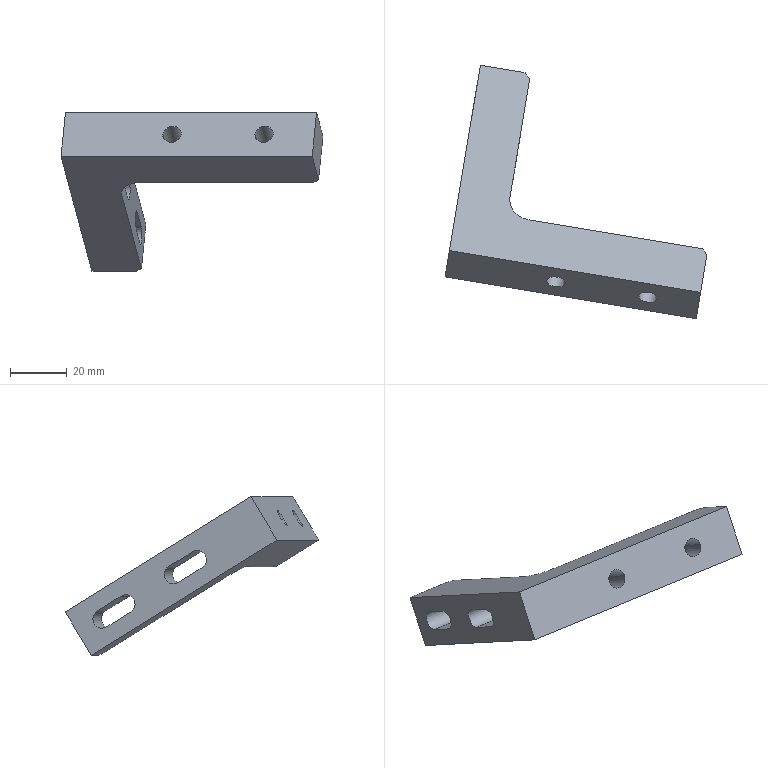Component | SolidWorks | 14AC-24-1-008-1 | 1 solid | 31 faces | box 92.56 x 89.67 x 56.08 mm | volume 43107 mm3 | plane 16 | cylinder 14 | spline 1 | commonest cylinder face diameters 6.6 x8 11 x4 16 x2
STEP:
#1=COLOUR_RGB('',0.7922,0.8196,0.9333);
#2=FILL_AREA_STYLE_COLOUR('',#1);
#3=FILL_AREA_STYLE('',(#2));
#4=SURFACE_STYLE_FILL_AREA(#3);
#5=SURFACE_SIDE_STYLE('',(#4));
#6=SURFACE_STYLE_USAGE(.BOTH.,#5);
#7=PRESENTATION_STYLE_ASSIGNMENT((#6));
#8=CARTESIAN_POINT('',(19.576,-9.025,-4.805));
#9=VERTEX_POINT('',#8);
#10=CARTESIAN_POINT('',(19.149,-8.954,-4.805));
#11=VERTEX_POINT('',#10);
#12=CARTESIAN_POINT('',(19.362,-8.99,-4.805));
#13=DIRECTION('',(0.1401,0.8413,-0.5222));
#14=DIRECTION('',(-0.9864,0.1642,0.));
#15=AXIS2_PLACEMENT_3D('',#12,#13,#14);
#16=CIRCLE('',#15,0.2165);
#17=EDGE_CURVE('',#9,#11,#16,.T.);
#18=ORIENTED_EDGE('',*,*,#17,.F.);
#19=CARTESIAN_POINT('',(19.613,-8.8,-4.944));
#20=VERTEX_POINT('',#19);
#21=CARTESIAN_POINT('',(19.613,-8.8,-4.944));
#22=DIRECTION('',(0.1401,0.8413,-0.5222));
#23=VECTOR('',#22,39.37);
#24=LINE('',#21,#23);
#25=EDGE_CURVE('',#9,#20,#24,.T.);
#26=ORIENTED_EDGE('',*,*,#25,.T.);
#27=CARTESIAN_POINT('',(19.186,-8.729,-4.944));
#28=VERTEX_POINT('',#27);
#29=CARTESIAN_POINT('',(19.4,-8.765,-4.944));
#30=DIRECTION('',(0.1401,0.8413,-0.5222));
#31=DIRECTION('',(-0.9864,0.1642,0.));
#32=AXIS2_PLACEMENT_3D('',#29,#30,#31);
#33=CIRCLE('',#32,0.2165);
#34=EDGE_CURVE('',#20,#28,#33,.T.);
#35=ORIENTED_EDGE('',*,*,#34,.T.);
#36=CARTESIAN_POINT('',(19.186,-8.729,-4.944));
#37=DIRECTION('',(0.1401,0.8413,-0.5222));
#38=VECTOR('',#37,39.37);
#39=LINE('',#36,#38);
#40=EDGE_CURVE('',#11,#28,#39,.T.);
#41=ORIENTED_EDGE('',*,*,#40,.F.);
#42=EDGE_LOOP('',(#18,#26,#35,#41));
#43=FACE_OUTER_BOUND('',#42,.T.);
#44=CARTESIAN_POINT('',(19.4,-8.765,-4.944));
#45=DIRECTION('',(0.1401,0.8413,-0.5222));
#46=DIRECTION('',(-0.9864,0.1642,0.));
#47=AXIS2_PLACEMENT_3D('',#44,#45,#46);
#48=CYLINDRICAL_SURFACE('',#47,0.2165);
#49=ADVANCED_FACE('',(#43),#48,.F.);
#50=CARTESIAN_POINT('',(19.429,-9.382,-4.574));
#51=VERTEX_POINT('',#50);
#52=CARTESIAN_POINT('',(19.172,-9.34,-4.574));
#53=VERTEX_POINT('',#52);
#54=CARTESIAN_POINT('',(19.301,-9.361,-4.574));
#55=DIRECTION('',(0.1401,0.8413,-0.5222));
#56=DIRECTION('',(-0.9864,0.1642,0.));
#57=AXIS2_PLACEMENT_3D('',#54,#55,#56);
#58=CIRCLE('',#57,0.1299);
#59=EDGE_CURVE('',#51,#53,#58,.T.);
#60=ORIENTED_EDGE('',*,*,#59,.F.);
#61=CARTESIAN_POINT('',(19.49,-9.011,-4.805));
#62=VERTEX_POINT('',#61);
#63=CARTESIAN_POINT('',(19.528,-8.786,-4.944));
#64=DIRECTION('',(0.1401,0.8413,-0.5222));
#65=VECTOR('',#64,39.37);
#66=LINE('',#63,#65);
#67=EDGE_CURVE('',#51,#62,#66,.T.);
#68=ORIENTED_EDGE('',*,*,#67,.T.);
#69=CARTESIAN_POINT('',(19.234,-8.969,-4.805));
#70=VERTEX_POINT('',#69);
#71=CARTESIAN_POINT('',(19.362,-8.99,-4.805));
#72=DIRECTION('',(0.1401,0.8413,-0.5222));
#73=DIRECTION('',(-0.9864,0.1642,0.));
#74=AXIS2_PLACEMENT_3D('',#71,#72,#73);
#75=CIRCLE('',#74,0.1299);
#76=EDGE_CURVE('',#62,#70,#75,.T.);
#77=ORIENTED_EDGE('',*,*,#76,.T.);
#78=CARTESIAN_POINT('',(19.272,-8.743,-4.944));
#79=DIRECTION('',(0.1401,0.8413,-0.5222));
#80=VECTOR('',#79,39.37);
#81=LINE('',#78,#80);
#82=EDGE_CURVE('',#53,#70,#81,.T.);
#83=ORIENTED_EDGE('',*,*,#82,.F.);
#84=EDGE_LOOP('',(#60,#68,#77,#83));
#85=FACE_OUTER_BOUND('',#84,.T.);
#86=CARTESIAN_POINT('',(19.4,-8.765,-4.944));
#87=DIRECTION('',(0.1401,0.8413,-0.5222));
#88=DIRECTION('',(-0.9864,0.1642,0.));
#89=AXIS2_PLACEMENT_3D('',#86,#87,#88);
#90=CYLINDRICAL_SURFACE('',#89,0.1299);
#91=ADVANCED_FACE('',(#85),#90,.F.);
#92=CARTESIAN_POINT('',(18.294,-8.812,-4.805));
#93=VERTEX_POINT('',#92);
#94=CARTESIAN_POINT('',(17.867,-8.741,-4.805));
#95=VERTEX_POINT('',#94);
#96=CARTESIAN_POINT('',(18.081,-8.776,-4.805));
#97=DIRECTION('',(0.1401,0.8413,-0.5222));
#98=DIRECTION('',(-0.9864,0.1642,0.));
#99=AXIS2_PLACEMENT_3D('',#96,#97,#98);
#100=CIRCLE('',#99,0.2165);
#101=EDGE_CURVE('',#93,#95,#100,.T.);
#102=ORIENTED_EDGE('',*,*,#101,.F.);
#103=CARTESIAN_POINT('',(18.332,-8.587,-4.944));
#104=VERTEX_POINT('',#103);
#105=CARTESIAN_POINT('',(18.332,-8.587,-4.944));
#106=DIRECTION('',(0.1401,0.8413,-0.5222));
#107=VECTOR('',#106,39.37);
#108=LINE('',#105,#107);
#109=EDGE_CURVE('',#93,#104,#108,.T.);
#110=ORIENTED_EDGE('',*,*,#109,.T.);
#111=CARTESIAN_POINT('',(17.905,-8.516,-4.944));
#112=VERTEX_POINT('',#111);
#113=CARTESIAN_POINT('',(18.118,-8.551,-4.944));
#114=DIRECTION('',(0.1401,0.8413,-0.5222));
#115=DIRECTION('',(-0.9864,0.1642,0.));
#116=AXIS2_PLACEMENT_3D('',#113,#114,#115);
#117=CIRCLE('',#116,0.2165);
#118=EDGE_CURVE('',#104,#112,#117,.T.);
#119=ORIENTED_EDGE('',*,*,#118,.T.);
#120=CARTESIAN_POINT('',(17.905,-8.516,-4.944));
#121=DIRECTION('',(0.1401,0.8413,-0.5222));
#122=VECTOR('',#121,39.37);
#123=LINE('',#120,#122);
#124=EDGE_CURVE('',#95,#112,#123,.T.);
#125=ORIENTED_EDGE('',*,*,#124,.F.);
#126=EDGE_LOOP('',(#102,#110,#119,#125));
#127=FACE_OUTER_BOUND('',#126,.T.);
#128=CARTESIAN_POINT('',(18.118,-8.551,-4.944));
#129=DIRECTION('',(0.1401,0.8413,-0.5222));
#130=DIRECTION('',(-0.9864,0.1642,0.));
#131=AXIS2_PLACEMENT_3D('',#128,#129,#130);
#132=CYLINDRICAL_SURFACE('',#131,0.2165);
#133=ADVANCED_FACE('',(#127),#132,.F.);
#134=CARTESIAN_POINT('',(18.147,-9.169,-4.574));
#135=VERTEX_POINT('',#134);
#136=CARTESIAN_POINT('',(17.891,-9.126,-4.574));
#137=VERTEX_POINT('',#136);
#138=CARTESIAN_POINT('',(18.019,-9.147,-4.574));
#139=DIRECTION('',(0.1401,0.8413,-0.5222));
#140=DIRECTION('',(-0.9864,0.1642,0.));
#141=AXIS2_PLACEMENT_3D('',#138,#139,#140);
#142=CIRCLE('',#141,0.1299);
#143=EDGE_CURVE('',#135,#137,#142,.T.);
#144=ORIENTED_EDGE('',*,*,#143,.F.);
#145=CARTESIAN_POINT('',(18.209,-8.798,-4.805));
#146=VERTEX_POINT('',#145);
#147=CARTESIAN_POINT('',(18.246,-8.573,-4.944));
#148=DIRECTION('',(0.1401,0.8413,-0.5222));
#149=VECTOR('',#148,39.37);
#150=LINE('',#147,#149);
#151=EDGE_CURVE('',#135,#146,#150,.T.);
#152=ORIENTED_EDGE('',*,*,#151,.T.);
#153=CARTESIAN_POINT('',(17.953,-8.755,-4.805));
#154=VERTEX_POINT('',#153);
#155=CARTESIAN_POINT('',(18.081,-8.776,-4.805));
#156=DIRECTION('',(0.1401,0.8413,-0.5222));
#157=DIRECTION('',(-0.9864,0.1642,0.));
#158=AXIS2_PLACEMENT_3D('',#155,#156,#157);
#159=CIRCLE('',#158,0.1299);
#160=EDGE_CURVE('',#146,#154,#159,.T.);
#161=ORIENTED_EDGE('',*,*,#160,.T.);
#162=CARTESIAN_POINT('',(17.99,-8.53,-4.944));
#163=DIRECTION('',(0.1401,0.8413,-0.5222));
#164=VECTOR('',#163,39.37);
#165=LINE('',#162,#164);
#166=EDGE_CURVE('',#137,#154,#165,.T.);
#167=ORIENTED_EDGE('',*,*,#166,.F.);
#168=EDGE_LOOP('',(#144,#152,#161,#167));
#169=FACE_OUTER_BOUND('',#168,.T.);
#170=CARTESIAN_POINT('',(18.118,-8.551,-4.944));
#171=DIRECTION('',(0.1401,0.8413,-0.5222));
#172=DIRECTION('',(-0.9864,0.1642,0.));
#173=AXIS2_PLACEMENT_3D('',#170,#171,#172);
#174=CYLINDRICAL_SURFACE('',#173,0.1299);
#175=ADVANCED_FACE('',(#169),#174,.F.);
#176=CARTESIAN_POINT('',(17.526,-6.598,-6.48));
#177=VERTEX_POINT('',#176);
#178=CARTESIAN_POINT('',(16.904,-6.494,-6.48));
#179=VERTEX_POINT('',#178);
#180=CARTESIAN_POINT('',(20.399,-7.076,-6.48));
#181=DIRECTION('',(-0.9864,0.1642,-0.));
#182=VECTOR('',#181,39.37);
#183=LINE('',#180,#182);
#184=EDGE_CURVE('',#177,#179,#183,.T.);
#185=ORIENTED_EDGE('',*,*,#184,.F.);
#186=CARTESIAN_POINT('',(17.592,-6.677,-6.439));
#187=VERTEX_POINT('',#186);
#188=CARTESIAN_POINT('',(17.526,-6.598,-6.48));
#189=DIRECTION('',(0.5985,-0.711,0.3692));
#190=VECTOR('',#189,39.37);
#191=LINE('',#188,#190);
#192=EDGE_CURVE('',#177,#187,#191,.T.);
#193=ORIENTED_EDGE('',*,*,#192,.T.);
#194=CARTESIAN_POINT('',(17.316,-8.333,-5.411));
#195=VERTEX_POINT('',#194);
#196=CARTESIAN_POINT('',(17.603,-6.611,-6.48));
#197=DIRECTION('',(0.1401,0.8413,-0.5222));
#198=VECTOR('',#197,39.37);
#199=LINE('',#196,#198);
#200=EDGE_CURVE('',#195,#187,#199,.T.);
#201=ORIENTED_EDGE('',*,*,#200,.F.);
#202=CARTESIAN_POINT('',(17.583,-8.65,-5.247));
#203=VERTEX_POINT('',#202);
#204=CARTESIAN_POINT('',(17.627,-8.385,-5.411));
#205=DIRECTION('',(0.08576,0.5151,0.8529));
#206=DIRECTION('',(-0.9864,0.1642,0.));
#207=AXIS2_PLACEMENT_3D('',#204,#205,#206);
#208=CIRCLE('',#207,0.315);
#209=EDGE_CURVE('',#195,#203,#208,.T.);
#210=ORIENTED_EDGE('',*,*,#209,.T.);
#211=CARTESIAN_POINT('',(19.991,-9.051,-5.247));
#212=VERTEX_POINT('',#211);
#213=CARTESIAN_POINT('',(20.068,-9.064,-5.247));
#214=DIRECTION('',(-0.9864,0.1642,-0.));
#215=VECTOR('',#214,39.37);
#216=LINE('',#213,#215);
#217=EDGE_CURVE('',#212,#203,#216,.T.);
#218=ORIENTED_EDGE('',*,*,#217,.F.);
#219=CARTESIAN_POINT('',(20.057,-9.13,-5.205));
#220=VERTEX_POINT('',#219);
#221=CARTESIAN_POINT('',(19.991,-9.051,-5.247));
#222=DIRECTION('',(0.5985,-0.711,0.3692));
#223=VECTOR('',#222,39.37);
#224=LINE('',#221,#223);
#225=EDGE_CURVE('',#212,#220,#224,.T.);
#226=ORIENTED_EDGE('',*,*,#225,.T.);
#227=CARTESIAN_POINT('',(19.969,-9.66,-4.877));
#228=VERTEX_POINT('',#227);
#229=CARTESIAN_POINT('',(20.399,-7.076,-6.48));
#230=DIRECTION('',(0.1401,0.8413,-0.5222));
#231=VECTOR('',#230,39.37);
#232=LINE('',#229,#231);
#233=EDGE_CURVE('',#228,#220,#232,.T.);
#234=ORIENTED_EDGE('',*,*,#233,.F.);
#235=CARTESIAN_POINT('',(16.474,-9.078,-4.877));
#236=VERTEX_POINT('',#235);
#237=CARTESIAN_POINT('',(19.969,-9.66,-4.877));
#238=DIRECTION('',(-0.9864,0.1642,-0.));
#239=VECTOR('',#238,39.37);
#240=LINE('',#237,#239);
#241=EDGE_CURVE('',#228,#236,#240,.T.);
#242=ORIENTED_EDGE('',*,*,#241,.T.);
#243=CARTESIAN_POINT('',(16.904,-6.494,-6.48));
#244=DIRECTION('',(0.1401,0.8413,-0.5222));
#245=VECTOR('',#244,39.37);
#246=LINE('',#243,#245);
#247=EDGE_CURVE('',#236,#179,#246,.T.);
#248=ORIENTED_EDGE('',*,*,#247,.T.);
#249=EDGE_LOOP('',(#185,#193,#201,#210,#218,#226,#234,#242,#248));
#250=FACE_OUTER_BOUND('',#249,.T.);
#251=CARTESIAN_POINT('',(20.399,-7.076,-6.48));
#252=DIRECTION('',(0.08576,0.5151,0.8529));
#253=DIRECTION('',(-0.9864,0.1642,-0.));
#254=AXIS2_PLACEMENT_3D('',#251,#252,#253);
#255=PLANE('',#254);
#256=ADVANCED_FACE('',(#250),#255,.F.);
#257=CARTESIAN_POINT('',(17.586,-6.233,-5.876));
#258=VERTEX_POINT('',#257);
#259=CARTESIAN_POINT('',(16.965,-6.129,-5.876));
#260=VERTEX_POINT('',#259);
#261=CARTESIAN_POINT('',(20.46,-6.711,-5.876));
#262=DIRECTION('',(-0.9864,0.1642,-0.));
#263=VECTOR('',#262,39.37);
#264=LINE('',#261,#263);
#265=EDGE_CURVE('',#258,#260,#264,.T.);
#266=ORIENTED_EDGE('',*,*,#265,.F.);
#267=CARTESIAN_POINT('',(17.526,-6.598,-6.48));
#268=DIRECTION('',(-0.08576,-0.5151,-0.8529));
#269=VECTOR('',#268,39.37);
#270=LINE('',#267,#269);
#271=EDGE_CURVE('',#258,#177,#270,.T.);
#272=ORIENTED_EDGE('',*,*,#271,.T.);
#273=ORIENTED_EDGE('',*,*,#184,.T.);
#274=CARTESIAN_POINT('',(16.904,-6.494,-6.48));
#275=DIRECTION('',(0.08576,0.5151,0.8529));
#276=VECTOR('',#275,39.37);
#277=LINE('',#274,#276);
#278=EDGE_CURVE('',#179,#260,#277,.T.);
#279=ORIENTED_EDGE('',*,*,#278,.T.);
#280=EDGE_LOOP('',(#266,#272,#273,#279));
#281=FACE_OUTER_BOUND('',#280,.T.);
#282=CARTESIAN_POINT('',(20.399,-7.076,-6.48));
#283=DIRECTION('',(-0.1401,-0.8413,0.5222));
#284=DIRECTION('',(0.9864,-0.1642,0.));
#285=AXIS2_PLACEMENT_3D('',#282,#283,#284);
#286=PLANE('',#285);
#287=ADVANCED_FACE('',(#281),#286,.F.);
#288=CARTESIAN_POINT('',(17.377,-7.968,-4.807));
#289=VERTEX_POINT('',#288);
#290=CARTESIAN_POINT('',(17.653,-6.312,-5.835));
#291=VERTEX_POINT('',#290);
#292=CARTESIAN_POINT('',(17.664,-6.246,-5.876));
#293=DIRECTION('',(0.1401,0.8413,-0.5222));
#294=VECTOR('',#293,39.37);
#295=LINE('',#292,#294);
#296=EDGE_CURVE('',#289,#291,#295,.T.);
#297=ORIENTED_EDGE('',*,*,#296,.T.);
#298=CARTESIAN_POINT('',(17.586,-6.233,-5.876));
#299=DIRECTION('',(-0.5985,0.711,-0.3692));
#300=VECTOR('',#299,39.37);
#301=LINE('',#298,#300);
#302=EDGE_CURVE('',#291,#258,#301,.T.);
#303=ORIENTED_EDGE('',*,*,#302,.T.);
#304=ORIENTED_EDGE('',*,*,#265,.T.);
#305=CARTESIAN_POINT('',(16.535,-8.713,-4.272));
#306=VERTEX_POINT('',#305);
#307=CARTESIAN_POINT('',(16.965,-6.129,-5.876));
#308=DIRECTION('',(-0.1401,-0.8413,0.5222));
#309=VECTOR('',#308,39.37);
#310=LINE('',#307,#309);
#311=EDGE_CURVE('',#260,#306,#310,.T.);
#312=ORIENTED_EDGE('',*,*,#311,.T.);
#313=CARTESIAN_POINT('',(20.03,-9.295,-4.272));
#314=VERTEX_POINT('',#313);
#315=CARTESIAN_POINT('',(20.03,-9.295,-4.272));
#316=DIRECTION('',(-0.9864,0.1642,-0.));
#317=VECTOR('',#316,39.37);
#318=LINE('',#315,#317);
#319=EDGE_CURVE('',#314,#306,#318,.T.);
#320=ORIENTED_EDGE('',*,*,#319,.F.);
#321=CARTESIAN_POINT('',(20.118,-8.765,-4.601));
#322=VERTEX_POINT('',#321);
#323=CARTESIAN_POINT('',(20.46,-6.711,-5.876));
#324=DIRECTION('',(-0.1401,-0.8413,0.5222));
#325=VECTOR('',#324,39.37);
#326=LINE('',#323,#325);
#327=EDGE_CURVE('',#322,#314,#326,.T.);
#328=ORIENTED_EDGE('',*,*,#327,.F.);
#329=CARTESIAN_POINT('',(20.052,-8.686,-4.642));
#330=VERTEX_POINT('',#329);
#331=CARTESIAN_POINT('',(20.052,-8.686,-4.642));
#332=DIRECTION('',(-0.5985,0.711,-0.3692));
#333=VECTOR('',#332,39.37);
#334=LINE('',#331,#333);
#335=EDGE_CURVE('',#322,#330,#334,.T.);
#336=ORIENTED_EDGE('',*,*,#335,.T.);
#337=CARTESIAN_POINT('',(17.644,-8.285,-4.642));
#338=VERTEX_POINT('',#337);
#339=CARTESIAN_POINT('',(20.129,-8.699,-4.642));
#340=DIRECTION('',(-0.9864,0.1642,-0.));
#341=VECTOR('',#340,39.37);
#342=LINE('',#339,#341);
#343=EDGE_CURVE('',#330,#338,#342,.T.);
#344=ORIENTED_EDGE('',*,*,#343,.T.);
#345=CARTESIAN_POINT('',(17.688,-8.02,-4.807));
#346=DIRECTION('',(-0.08576,-0.5151,-0.8529));
#347=DIRECTION('',(0.9864,-0.1642,0.));
#348=AXIS2_PLACEMENT_3D('',#345,#346,#347);
#349=CIRCLE('',#348,0.315);
#350=EDGE_CURVE('',#338,#289,#349,.T.);
#351=ORIENTED_EDGE('',*,*,#350,.T.);
#352=EDGE_LOOP('',(#297,#303,#304,#312,#320,#328,#336,#344,#351));
#353=FACE_OUTER_BOUND('',#352,.T.);
#354=CARTESIAN_POINT('',(20.46,-6.711,-5.876));
#355=DIRECTION('',(-0.08576,-0.5151,-0.8529));
#356=DIRECTION('',(0.9864,-0.1642,0.));
#357=AXIS2_PLACEMENT_3D('',#354,#355,#356);
#358=PLANE('',#357);
#359=ADVANCED_FACE('',(#353),#358,.F.);
#360=CARTESIAN_POINT('',(19.301,-9.361,-4.574));
#361=DIRECTION('',(0.1401,0.8413,-0.5222));
#362=DIRECTION('',(-0.9864,0.1642,0.));
#363=AXIS2_PLACEMENT_3D('',#360,#361,#362);
#364=CIRCLE('',#363,0.1299);
#365=EDGE_CURVE('',#53,#51,#364,.T.);
#366=ORIENTED_EDGE('',*,*,#365,.T.);
#367=ORIENTED_EDGE('',*,*,#59,.T.);
#368=EDGE_LOOP('',(#366,#367));
#369=FACE_BOUND('',#368,.T.);
#370=CARTESIAN_POINT('',(18.019,-9.147,-4.574));
#371=DIRECTION('',(0.1401,0.8413,-0.5222));
#372=DIRECTION('',(-0.9864,0.1642,0.));
#373=AXIS2_PLACEMENT_3D('',#370,#371,#372);
#374=CIRCLE('',#373,0.1299);
#375=EDGE_CURVE('',#137,#135,#374,.T.);
#376=ORIENTED_EDGE('',*,*,#375,.T.);
#377=ORIENTED_EDGE('',*,*,#143,.T.);
#378=EDGE_LOOP('',(#376,#377));
#379=FACE_BOUND('',#378,.T.);
#380=CARTESIAN_POINT('',(16.474,-9.078,-4.877));
#381=DIRECTION('',(-0.08576,-0.5151,-0.8529));
#382=VECTOR('',#381,39.37);
#383=LINE('',#380,#382);
#384=EDGE_CURVE('',#306,#236,#383,.T.);
#385=ORIENTED_EDGE('',*,*,#384,.T.);
#386=ORIENTED_EDGE('',*,*,#241,.F.);
#387=CARTESIAN_POINT('',(19.969,-9.66,-4.877));
#388=DIRECTION('',(-0.08576,-0.5151,-0.8529));
#389=VECTOR('',#388,39.37);
#390=LINE('',#387,#389);
#391=EDGE_CURVE('',#314,#228,#390,.T.);
#392=ORIENTED_EDGE('',*,*,#391,.F.);
#393=ORIENTED_EDGE('',*,*,#319,.T.);
#394=EDGE_LOOP('',(#385,#386,#392,#393));
#395=FACE_OUTER_BOUND('',#394,.T.);
#396=CARTESIAN_POINT('',(19.969,-9.66,-4.877));
#397=DIRECTION('',(0.1401,0.8413,-0.5222));
#398=DIRECTION('',(-0.9864,0.1642,-0.));
#399=AXIS2_PLACEMENT_3D('',#396,#397,#398);
#400=PLANE('',#399);
#401=ADVANCED_FACE('',(#369,#379,#395),#400,.F.);
#402=ORIENTED_EDGE('',*,*,#233,.T.);
#403=CARTESIAN_POINT('',(20.057,-9.13,-5.205));
#404=DIRECTION('',(0.08576,0.5151,0.8529));
#405=VECTOR('',#404,39.37);
#406=LINE('',#403,#405);
#407=EDGE_CURVE('',#220,#322,#406,.T.);
#408=ORIENTED_EDGE('',*,*,#407,.T.);
#409=ORIENTED_EDGE('',*,*,#327,.T.);
#410=ORIENTED_EDGE('',*,*,#391,.T.);
#411=EDGE_LOOP('',(#402,#408,#409,#410));
#412=FACE_OUTER_BOUND('',#411,.T.);
#413=CARTESIAN_POINT('',(19.969,-9.66,-4.877));
#414=DIRECTION('',(-0.9864,0.1642,-0.));
#415=DIRECTION('',(-0.08576,-0.5151,-0.8529));
#416=AXIS2_PLACEMENT_3D('',#413,#414,#415);
#417=PLANE('',#416);
#418=ADVANCED_FACE('',(#412),#417,.F.);
#419=CARTESIAN_POINT('',(16.725,-7.57,-5.245));
#420=VERTEX_POINT('',#419);
#421=CARTESIAN_POINT('',(16.703,-7.704,-5.466));
#422=VERTEX_POINT('',#421);
#423=CARTESIAN_POINT('',(16.714,-7.637,-5.356));
#424=DIRECTION('',(-0.9864,0.1642,-0.));
#425=DIRECTION('',(-0.08576,-0.5151,-0.8529));
#426=AXIS2_PLACEMENT_3D('',#423,#424,#425);
#427=CIRCLE('',#426,0.1299);
#428=EDGE_CURVE('',#420,#422,#427,.T.);
#429=ORIENTED_EDGE('',*,*,#428,.F.);
#430=CARTESIAN_POINT('',(16.67,-7.901,-5.039));
#431=VERTEX_POINT('',#430);
#432=CARTESIAN_POINT('',(16.725,-7.57,-5.245));
#433=DIRECTION('',(0.1401,0.8413,-0.5222));
#434=VECTOR('',#433,39.37);
#435=LINE('',#432,#434);
#436=EDGE_CURVE('',#431,#420,#435,.T.);
#437=ORIENTED_EDGE('',*,*,#436,.F.);
#438=CARTESIAN_POINT('',(16.648,-8.035,-5.261));
#439=VERTEX_POINT('',#438);
#440=CARTESIAN_POINT('',(16.659,-7.968,-5.15));
#441=DIRECTION('',(-0.9864,0.1642,-0.));
#442=DIRECTION('',(-0.08576,-0.5151,-0.8529));
#443=AXIS2_PLACEMENT_3D('',#440,#441,#442);
#444=CIRCLE('',#443,0.1299);
#445=EDGE_CURVE('',#439,#431,#444,.T.);
#446=ORIENTED_EDGE('',*,*,#445,.F.);
#447=CARTESIAN_POINT('',(16.703,-7.704,-5.466));
#448=DIRECTION('',(-0.1401,-0.8413,0.5222));
#449=VECTOR('',#448,39.37);
#450=LINE('',#447,#449);
#451=EDGE_CURVE('',#422,#439,#450,.T.);
#452=ORIENTED_EDGE('',*,*,#451,.F.);
#453=EDGE_LOOP('',(#429,#437,#446,#452));
#454=FACE_BOUND('',#453,.T.);
#455=CARTESIAN_POINT('',(16.891,-6.576,-5.861));
#456=VERTEX_POINT('',#455);
#457=CARTESIAN_POINT('',(16.868,-6.71,-6.083));
#458=VERTEX_POINT('',#457);
#459=CARTESIAN_POINT('',(16.879,-6.643,-5.972));
#460=DIRECTION('',(-0.9864,0.1642,-0.));
#461=DIRECTION('',(-0.08576,-0.5151,-0.8529));
#462=AXIS2_PLACEMENT_3D('',#459,#460,#461);
#463=CIRCLE('',#462,0.1299);
#464=EDGE_CURVE('',#456,#458,#463,.T.);
#465=ORIENTED_EDGE('',*,*,#464,.F.);
#466=CARTESIAN_POINT('',(16.835,-6.907,-5.656));
#467=VERTEX_POINT('',#466);
#468=CARTESIAN_POINT('',(16.891,-6.576,-5.861));
#469=DIRECTION('',(0.1401,0.8413,-0.5222));
#470=VECTOR('',#469,39.37);
#471=LINE('',#468,#470);
#472=EDGE_CURVE('',#467,#456,#471,.T.);
#473=ORIENTED_EDGE('',*,*,#472,.F.);
#474=CARTESIAN_POINT('',(16.813,-7.041,-5.877));
#475=VERTEX_POINT('',#474);
#476=CARTESIAN_POINT('',(16.824,-6.974,-5.767));
#477=DIRECTION('',(-0.9864,0.1642,-0.));
#478=DIRECTION('',(-0.08576,-0.5151,-0.8529));
#479=AXIS2_PLACEMENT_3D('',#476,#477,#478);
#480=CIRCLE('',#479,0.1299);
#481=EDGE_CURVE('',#475,#467,#480,.T.);
#482=ORIENTED_EDGE('',*,*,#481,.F.);
#483=CARTESIAN_POINT('',(16.868,-6.71,-6.083));
#484=DIRECTION('',(-0.1401,-0.8413,0.5222));
#485=VECTOR('',#484,39.37);
#486=LINE('',#483,#485);
#487=EDGE_CURVE('',#458,#475,#486,.T.);
#488=ORIENTED_EDGE('',*,*,#487,.F.);
#489=EDGE_LOOP('',(#465,#473,#482,#488));
#490=FACE_BOUND('',#489,.T.);
#491=ORIENTED_EDGE('',*,*,#247,.F.);
#492=ORIENTED_EDGE('',*,*,#384,.F.);
#493=ORIENTED_EDGE('',*,*,#311,.F.);
#494=ORIENTED_EDGE('',*,*,#278,.F.);
#495=EDGE_LOOP('',(#491,#492,#493,#494));
#496=FACE_OUTER_BOUND('',#495,.T.);
#497=CARTESIAN_POINT('',(16.474,-9.078,-4.877));
#498=DIRECTION('',(-0.9864,0.1642,-0.));
#499=DIRECTION('',(-0.08576,-0.5151,-0.8529));
#500=AXIS2_PLACEMENT_3D('',#497,#498,#499);
#501=PLANE('',#500);
#502=ADVANCED_FACE('',(#454,#490,#496),#501,.T.);
#503=ORIENTED_EDGE('',*,*,#200,.T.);
#504=CARTESIAN_POINT('',(17.653,-6.312,-5.835));
#505=DIRECTION('',(0.08576,0.5151,0.8529));
#506=VECTOR('',#505,39.37);
#507=LINE('',#504,#506);
#508=EDGE_CURVE('',#187,#291,#507,.T.);
#509=ORIENTED_EDGE('',*,*,#508,.T.);
#510=ORIENTED_EDGE('',*,*,#296,.F.);
#511=CARTESIAN_POINT('',(17.356,-8.097,-5.021));
#512=VERTEX_POINT('',#511);
#513=CARTESIAN_POINT('',(17.316,-8.333,-5.411));
#514=DIRECTION('',(-0.08576,-0.5151,-0.8529));
#515=VECTOR('',#514,39.37);
#516=LINE('',#513,#515);
#517=EDGE_CURVE('',#289,#512,#516,.T.);
#518=ORIENTED_EDGE('',*,*,#517,.T.);
#519=CARTESIAN_POINT('',(17.369,-8.017,-5.039));
#520=VERTEX_POINT('',#519);
#521=CARTESIAN_POINT('',(17.358,-8.084,-5.15));
#522=DIRECTION('',(-0.9864,0.1642,-0.));
#523=DIRECTION('',(-0.1401,-0.8413,0.5222));
#524=AXIS2_PLACEMENT_3D('',#521,#522,#523);
#525=CIRCLE('',#524,0.1299);
#526=EDGE_CURVE('',#512,#520,#525,.T.);
#527=ORIENTED_EDGE('',*,*,#526,.T.);
#528=CARTESIAN_POINT('',(17.424,-7.686,-5.245));
#529=VERTEX_POINT('',#528);
#530=CARTESIAN_POINT('',(17.645,-6.361,-6.067));
#531=DIRECTION('',(0.1401,0.8413,-0.5222));
#532=VECTOR('',#531,39.37);
#533=LINE('',#530,#532);
#534=EDGE_CURVE('',#520,#529,#533,.T.);
#535=ORIENTED_EDGE('',*,*,#534,.T.);
#536=CARTESIAN_POINT('',(17.402,-7.82,-5.466));
#537=VERTEX_POINT('',#536);
#538=CARTESIAN_POINT('',(17.413,-7.753,-5.356));
#539=DIRECTION('',(-0.9864,0.1642,-0.));
#540=DIRECTION('',(-0.1401,-0.8413,0.5222));
#541=AXIS2_PLACEMENT_3D('',#538,#539,#540);
#542=CIRCLE('',#541,0.1299);
#543=EDGE_CURVE('',#529,#537,#542,.T.);
#544=ORIENTED_EDGE('',*,*,#543,.T.);
#545=CARTESIAN_POINT('',(17.347,-8.151,-5.261));
#546=VERTEX_POINT('',#545);
#547=CARTESIAN_POINT('',(17.622,-6.495,-6.289));
#548=DIRECTION('',(-0.1401,-0.8413,0.5222));
#549=VECTOR('',#548,39.37);
#550=LINE('',#547,#549);
#551=EDGE_CURVE('',#537,#546,#550,.T.);
#552=ORIENTED_EDGE('',*,*,#551,.T.);
#553=CARTESIAN_POINT('',(17.338,-8.204,-5.197));
#554=VERTEX_POINT('',#553);
#555=CARTESIAN_POINT('',(17.358,-8.084,-5.15));
#556=DIRECTION('',(-0.9864,0.1642,-0.));
#557=DIRECTION('',(-0.1401,-0.8413,0.5222));
#558=AXIS2_PLACEMENT_3D('',#555,#556,#557);
#559=CIRCLE('',#558,0.1299);
#560=EDGE_CURVE('',#546,#554,#559,.T.);
#561=ORIENTED_EDGE('',*,*,#560,.T.);
#562=CARTESIAN_POINT('',(17.316,-8.333,-5.411));
#563=DIRECTION('',(-0.08576,-0.5151,-0.8529));
#564=VECTOR('',#563,39.37);
#565=LINE('',#562,#564);
#566=EDGE_CURVE('',#554,#195,#565,.T.);
#567=ORIENTED_EDGE('',*,*,#566,.T.);
#568=EDGE_LOOP('',(#503,#509,#510,#518,#527,#535,#544,#552,#561,#567));
#569=FACE_OUTER_BOUND('',#568,.T.);
#570=CARTESIAN_POINT('',(17.534,-7.024,-5.656));
#571=VERTEX_POINT('',#570);
#572=CARTESIAN_POINT('',(17.59,-6.693,-5.861));
#573=VERTEX_POINT('',#572);
#574=CARTESIAN_POINT('',(17.645,-6.361,-6.067));
#575=DIRECTION('',(0.1401,0.8413,-0.5222));
#576=VECTOR('',#575,39.37);
#577=LINE('',#574,#576);
#578=EDGE_CURVE('',#571,#573,#577,.T.);
#579=ORIENTED_EDGE('',*,*,#578,.T.);
#580=CARTESIAN_POINT('',(17.567,-6.826,-6.083));
#581=VERTEX_POINT('',#580);
#582=CARTESIAN_POINT('',(17.578,-6.759,-5.972));
#583=DIRECTION('',(-0.9864,0.1642,-0.));
#584=DIRECTION('',(-0.1401,-0.8413,0.5222));
#585=AXIS2_PLACEMENT_3D('',#582,#583,#584);
#586=CIRCLE('',#585,0.1299);
#587=EDGE_CURVE('',#573,#581,#586,.T.);
#588=ORIENTED_EDGE('',*,*,#587,.T.);
#589=CARTESIAN_POINT('',(17.512,-7.158,-5.877));
#590=VERTEX_POINT('',#589);
#591=CARTESIAN_POINT('',(17.622,-6.495,-6.289));
#592=DIRECTION('',(-0.1401,-0.8413,0.5222));
#593=VECTOR('',#592,39.37);
#594=LINE('',#591,#593);
#595=EDGE_CURVE('',#581,#590,#594,.T.);
#596=ORIENTED_EDGE('',*,*,#595,.T.);
#597=CARTESIAN_POINT('',(17.523,-7.091,-5.767));
#598=DIRECTION('',(-0.9864,0.1642,-0.));
#599=DIRECTION('',(-0.1401,-0.8413,0.5222));
#600=AXIS2_PLACEMENT_3D('',#597,#598,#599);
#601=CIRCLE('',#600,0.1299);
#602=EDGE_CURVE('',#590,#571,#601,.T.);
#603=ORIENTED_EDGE('',*,*,#602,.T.);
#604=EDGE_LOOP('',(#579,#588,#596,#603));
#605=FACE_BOUND('',#604,.T.);
#606=CARTESIAN_POINT('',(17.664,-6.246,-5.876));
#607=DIRECTION('',(-0.9864,0.1642,-0.));
#608=DIRECTION('',(-0.1401,-0.8413,0.5222));
#609=AXIS2_PLACEMENT_3D('',#606,#607,#608);
#610=PLANE('',#609);
#611=ADVANCED_FACE('',(#569,#605),#610,.F.);
#612=CARTESIAN_POINT('',(19.4,-8.765,-4.944));
#613=DIRECTION('',(0.1401,0.8413,-0.5222));
#614=DIRECTION('',(-0.9864,0.1642,0.));
#615=AXIS2_PLACEMENT_3D('',#612,#613,#614);
#616=CIRCLE('',#615,0.2165);
#617=EDGE_CURVE('',#28,#20,#616,.T.);
#618=ORIENTED_EDGE('',*,*,#617,.F.);
#619=ORIENTED_EDGE('',*,*,#34,.F.);
#620=EDGE_LOOP('',(#618,#619));
#621=FACE_BOUND('',#620,.T.);
#622=CARTESIAN_POINT('',(18.118,-8.551,-4.944));
#623=DIRECTION('',(0.1401,0.8413,-0.5222));
#624=DIRECTION('',(-0.9864,0.1642,0.));
#625=AXIS2_PLACEMENT_3D('',#622,#623,#624);
#626=CIRCLE('',#625,0.2165);
#627=EDGE_CURVE('',#112,#104,#626,.T.);
#628=ORIENTED_EDGE('',*,*,#627,.F.);
#629=ORIENTED_EDGE('',*,*,#118,.F.);
#630=EDGE_LOOP('',(#628,#629));
#631=FACE_BOUND('',#630,.T.);
#632=ORIENTED_EDGE('',*,*,#343,.F.);
#633=CARTESIAN_POINT('',(20.052,-8.686,-4.642));
#634=DIRECTION('',(-0.08576,-0.5151,-0.8529));
#635=VECTOR('',#634,39.37);
#636=LINE('',#633,#635);
#637=EDGE_CURVE('',#330,#212,#636,.T.);
#638=ORIENTED_EDGE('',*,*,#637,.T.);
#639=ORIENTED_EDGE('',*,*,#217,.T.);
#640=CARTESIAN_POINT('',(17.604,-8.52,-5.033));
#641=VERTEX_POINT('',#640);
#642=CARTESIAN_POINT('',(17.644,-8.285,-4.642));
#643=DIRECTION('',(0.08576,0.5151,0.8529));
#644=VECTOR('',#643,39.37);
#645=LINE('',#642,#644);
#646=EDGE_CURVE('',#203,#641,#645,.T.);
#647=ORIENTED_EDGE('',*,*,#646,.T.);
#648=CARTESIAN_POINT('',(17.622,-8.414,-4.856));
#649=VERTEX_POINT('',#648);
#650=CARTESIAN_POINT('',(17.604,-8.52,-5.033));
#651=CARTESIAN_POINT('',(17.606,-8.512,-5.018));
#652=CARTESIAN_POINT('',(17.606,-8.503,-5.003));
#653=CARTESIAN_POINT('',(17.607,-8.484,-4.974));
#654=CARTESIAN_POINT('',(17.608,-8.475,-4.959));
#655=CARTESIAN_POINT('',(17.611,-8.458,-4.93));
#656=CARTESIAN_POINT('',(17.613,-8.449,-4.915));
#657=CARTESIAN_POINT('',(17.618,-8.432,-4.886));
#658=CARTESIAN_POINT('',(17.621,-8.423,-4.871));
#659=CARTESIAN_POINT('',(17.622,-8.414,-4.856));
#660=B_SPLINE_CURVE_WITH_KNOTS('',3,(#650,#651,#652,#653,#654,#655,#656,#657,#658,#659),.UNSPECIFIED.,.F.,.F.,(4,2,2,2,4),(0.,0.001312,0.002624,0.003936,0.005248),.UNSPECIFIED.);
#661=EDGE_CURVE('',#641,#649,#660,.T.);
#662=ORIENTED_EDGE('',*,*,#661,.T.);
#663=CARTESIAN_POINT('',(17.644,-8.285,-4.642));
#664=DIRECTION('',(0.08576,0.5151,0.8529));
#665=VECTOR('',#664,39.37);
#666=LINE('',#663,#665);
#667=EDGE_CURVE('',#649,#338,#666,.T.);
#668=ORIENTED_EDGE('',*,*,#667,.T.);
#669=EDGE_LOOP('',(#632,#638,#639,#647,#662,#668));
#670=FACE_OUTER_BOUND('',#669,.T.);
#671=CARTESIAN_POINT('',(20.129,-8.699,-4.642));
#672=DIRECTION('',(-0.1401,-0.8413,0.5222));
#673=DIRECTION('',(0.9864,-0.1642,0.));
#674=AXIS2_PLACEMENT_3D('',#671,#672,#673);
#675=PLANE('',#674);
#676=ADVANCED_FACE('',(#621,#631,#670),#675,.F.);
#677=CARTESIAN_POINT('',(20.386,-7.158,-5.861));
#678=DIRECTION('',(-0.9864,0.1642,-0.));
#679=VECTOR('',#678,39.37);
#680=LINE('',#677,#679);
#681=EDGE_CURVE('',#573,#456,#680,.T.);
#682=ORIENTED_EDGE('',*,*,#681,.T.);
#683=ORIENTED_EDGE('',*,*,#464,.T.);
#684=CARTESIAN_POINT('',(20.363,-7.292,-6.083));
#685=DIRECTION('',(-0.9864,0.1642,-0.));
#686=VECTOR('',#685,39.37);
#687=LINE('',#684,#686);
#688=EDGE_CURVE('',#581,#458,#687,.T.);
#689=ORIENTED_EDGE('',*,*,#688,.F.);
#690=ORIENTED_EDGE('',*,*,#587,.F.);
#691=EDGE_LOOP('',(#682,#683,#689,#690));
#692=FACE_OUTER_BOUND('',#691,.T.);
#693=CARTESIAN_POINT('',(20.375,-7.225,-5.972));
#694=DIRECTION('',(-0.9864,0.1642,-0.));
#695=DIRECTION('',(-0.08576,-0.5151,-0.8529));
#696=AXIS2_PLACEMENT_3D('',#693,#694,#695);
#697=CYLINDRICAL_SURFACE('',#696,0.1299);
#698=ADVANCED_FACE('',(#692),#697,.F.);
#699=CARTESIAN_POINT('',(20.331,-7.489,-5.656));
#700=DIRECTION('',(-0.9864,0.1642,-0.));
#701=VECTOR('',#700,39.37);
#702=LINE('',#699,#701);
#703=EDGE_CURVE('',#571,#467,#702,.T.);
#704=ORIENTED_EDGE('',*,*,#703,.T.);
#705=ORIENTED_EDGE('',*,*,#472,.T.);
#706=ORIENTED_EDGE('',*,*,#681,.F.);
#707=ORIENTED_EDGE('',*,*,#578,.F.);
#708=EDGE_LOOP('',(#704,#705,#706,#707));
#709=FACE_OUTER_BOUND('',#708,.T.);
#710=CARTESIAN_POINT('',(20.386,-7.158,-5.861));
#711=DIRECTION('',(0.08576,0.5151,0.8529));
#712=DIRECTION('',(-0.9864,0.1642,-0.));
#713=AXIS2_PLACEMENT_3D('',#710,#711,#712);
#714=PLANE('',#713);
#715=ADVANCED_FACE('',(#709),#714,.F.);
#716=CARTESIAN_POINT('',(20.308,-7.623,-5.877));
#717=DIRECTION('',(-0.9864,0.1642,-0.));
#718=VECTOR('',#717,39.37);
#719=LINE('',#716,#718);
#720=EDGE_CURVE('',#590,#475,#719,.T.);
#721=ORIENTED_EDGE('',*,*,#720,.T.);
#722=ORIENTED_EDGE('',*,*,#481,.T.);
#723=ORIENTED_EDGE('',*,*,#703,.F.);
#724=ORIENTED_EDGE('',*,*,#602,.F.);
#725=EDGE_LOOP('',(#721,#722,#723,#724));
#726=FACE_OUTER_BOUND('',#725,.T.);
#727=CARTESIAN_POINT('',(20.319,-7.556,-5.767));
#728=DIRECTION('',(-0.9864,0.1642,-0.));
#729=DIRECTION('',(-0.08576,-0.5151,-0.8529));
#730=AXIS2_PLACEMENT_3D('',#727,#728,#729);
#731=CYLINDRICAL_SURFACE('',#730,0.1299);
#732=ADVANCED_FACE('',(#726),#731,.F.);
#733=ORIENTED_EDGE('',*,*,#688,.T.);
#734=ORIENTED_EDGE('',*,*,#487,.T.);
#735=ORIENTED_EDGE('',*,*,#720,.F.);
#736=ORIENTED_EDGE('',*,*,#595,.F.);
#737=EDGE_LOOP('',(#733,#734,#735,#736));
#738=FACE_OUTER_BOUND('',#737,.T.);
#739=CARTESIAN_POINT('',(20.363,-7.292,-6.083));
#740=DIRECTION('',(-0.08576,-0.5151,-0.8529));
#741=DIRECTION('',(0.1401,0.8413,-0.5222));
#742=AXIS2_PLACEMENT_3D('',#739,#740,#741);
#743=PLANE('',#742);
#744=ADVANCED_FACE('',(#738),#743,.F.);
#745=CARTESIAN_POINT('',(20.22,-8.152,-5.245));
#746=DIRECTION('',(-0.9864,0.1642,-0.));
#747=VECTOR('',#746,39.37);
#748=LINE('',#745,#747);
#749=EDGE_CURVE('',#529,#420,#748,.T.);
#750=ORIENTED_EDGE('',*,*,#749,.T.);
#751=ORIENTED_EDGE('',*,*,#428,.T.);
#752=CARTESIAN_POINT('',(20.198,-8.286,-5.466));
#753=DIRECTION('',(-0.9864,0.1642,-0.));
#754=VECTOR('',#753,39.37);
#755=LINE('',#752,#754);
#756=EDGE_CURVE('',#537,#422,#755,.T.);
#757=ORIENTED_EDGE('',*,*,#756,.F.);
#758=ORIENTED_EDGE('',*,*,#543,.F.);
#759=EDGE_LOOP('',(#750,#751,#757,#758));
#760=FACE_OUTER_BOUND('',#759,.T.);
#761=CARTESIAN_POINT('',(20.209,-8.219,-5.356));
#762=DIRECTION('',(-0.9864,0.1642,-0.));
#763=DIRECTION('',(-0.08576,-0.5151,-0.8529));
#764=AXIS2_PLACEMENT_3D('',#761,#762,#763);
#765=CYLINDRICAL_SURFACE('',#764,0.1299);
#766=ADVANCED_FACE('',(#760),#765,.F.);
#767=CARTESIAN_POINT('',(20.165,-8.483,-5.039));
#768=DIRECTION('',(-0.9864,0.1642,-0.));
#769=VECTOR('',#768,39.37);
#770=LINE('',#767,#769);
#771=EDGE_CURVE('',#520,#431,#770,.T.);
#772=ORIENTED_EDGE('',*,*,#771,.T.);
#773=ORIENTED_EDGE('',*,*,#436,.T.);
#774=ORIENTED_EDGE('',*,*,#749,.F.);
#775=ORIENTED_EDGE('',*,*,#534,.F.);
#776=EDGE_LOOP('',(#772,#773,#774,#775));
#777=FACE_OUTER_BOUND('',#776,.T.);
#778=CARTESIAN_POINT('',(20.22,-8.152,-5.245));
#779=DIRECTION('',(0.08576,0.5151,0.8529));
#780=DIRECTION('',(-0.9864,0.1642,-0.));
#781=AXIS2_PLACEMENT_3D('',#778,#779,#780);
#782=PLANE('',#781);
#783=ADVANCED_FACE('',(#777),#782,.F.);
#784=CARTESIAN_POINT('',(20.143,-8.617,-5.261));
#785=DIRECTION('',(-0.9864,0.1642,-0.));
#786=VECTOR('',#785,39.37);
#787=LINE('',#784,#786);
#788=EDGE_CURVE('',#546,#439,#787,.T.);
#789=ORIENTED_EDGE('',*,*,#788,.T.);
#790=ORIENTED_EDGE('',*,*,#445,.T.);
#791=ORIENTED_EDGE('',*,*,#771,.F.);
#792=ORIENTED_EDGE('',*,*,#526,.F.);
#793=CARTESIAN_POINT('',(17.358,-8.084,-5.15));
#794=DIRECTION('',(-0.9864,0.1642,-0.));
#795=DIRECTION('',(-0.1401,-0.8413,0.5222));
#796=AXIS2_PLACEMENT_3D('',#793,#794,#795);
#797=CIRCLE('',#796,0.1299);
#798=EDGE_CURVE('',#554,#512,#797,.T.);
#799=ORIENTED_EDGE('',*,*,#798,.F.);
#800=ORIENTED_EDGE('',*,*,#560,.F.);
#801=EDGE_LOOP('',(#789,#790,#791,#792,#799,#800));
#802=FACE_OUTER_BOUND('',#801,.T.);
#803=CARTESIAN_POINT('',(20.154,-8.55,-5.15));
#804=DIRECTION('',(-0.9864,0.1642,-0.));
#805=DIRECTION('',(-0.08576,-0.5151,-0.8529));
#806=AXIS2_PLACEMENT_3D('',#803,#804,#805);
#807=CYLINDRICAL_SURFACE('',#806,0.1299);
#808=ADVANCED_FACE('',(#802),#807,.F.);
#809=ORIENTED_EDGE('',*,*,#756,.T.);
#810=ORIENTED_EDGE('',*,*,#451,.T.);
#811=ORIENTED_EDGE('',*,*,#788,.F.);
#812=ORIENTED_EDGE('',*,*,#551,.F.);
#813=EDGE_LOOP('',(#809,#810,#811,#812));
#814=FACE_OUTER_BOUND('',#813,.T.);
#815=CARTESIAN_POINT('',(20.198,-8.286,-5.466));
#816=DIRECTION('',(-0.08576,-0.5151,-0.8529));
#817=DIRECTION('',(0.1401,0.8413,-0.5222));
#818=AXIS2_PLACEMENT_3D('',#815,#816,#817);
#819=PLANE('',#818);
#820=ADVANCED_FACE('',(#814),#819,.F.);
#821=ORIENTED_EDGE('',*,*,#151,.F.);
#822=ORIENTED_EDGE('',*,*,#375,.F.);
#823=ORIENTED_EDGE('',*,*,#166,.T.);
#824=CARTESIAN_POINT('',(18.081,-8.776,-4.805));
#825=DIRECTION('',(0.1401,0.8413,-0.5222));
#826=DIRECTION('',(-0.9864,0.1642,0.));
#827=AXIS2_PLACEMENT_3D('',#824,#825,#826);
#828=CIRCLE('',#827,0.1299);
#829=EDGE_CURVE('',#154,#146,#828,.T.);
#830=ORIENTED_EDGE('',*,*,#829,.T.);
#831=EDGE_LOOP('',(#821,#822,#823,#830));
#832=FACE_OUTER_BOUND('',#831,.T.);
#833=CARTESIAN_POINT('',(18.118,-8.551,-4.944));
#834=DIRECTION('',(0.1401,0.8413,-0.5222));
#835=DIRECTION('',(-0.9864,0.1642,0.));
#836=AXIS2_PLACEMENT_3D('',#833,#834,#835);
#837=CYLINDRICAL_SURFACE('',#836,0.1299);
#838=ADVANCED_FACE('',(#832),#837,.F.);
#839=ORIENTED_EDGE('',*,*,#829,.F.);
#840=ORIENTED_EDGE('',*,*,#160,.F.);
#841=EDGE_LOOP('',(#839,#840));
#842=FACE_BOUND('',#841,.T.);
#843=CARTESIAN_POINT('',(18.081,-8.776,-4.805));
#844=DIRECTION('',(0.1401,0.8413,-0.5222));
#845=DIRECTION('',(-0.9864,0.1642,0.));
#846=AXIS2_PLACEMENT_3D('',#843,#844,#845);
#847=CIRCLE('',#846,0.2165);
#848=EDGE_CURVE('',#95,#93,#847,.T.);
#849=ORIENTED_EDGE('',*,*,#848,.T.);
#850=ORIENTED_EDGE('',*,*,#101,.T.);
#851=EDGE_LOOP('',(#849,#850));
#852=FACE_OUTER_BOUND('',#851,.T.);
#853=CARTESIAN_POINT('',(18.092,-8.71,-4.694));
#854=DIRECTION('',(-0.1401,-0.8413,0.5222));
#855=DIRECTION('',(0.9864,-0.1642,0.));
#856=AXIS2_PLACEMENT_3D('',#853,#854,#855);
#857=PLANE('',#856);
#858=ADVANCED_FACE('',(#842,#852),#857,.F.);
#859=ORIENTED_EDGE('',*,*,#109,.F.);
#860=ORIENTED_EDGE('',*,*,#848,.F.);
#861=ORIENTED_EDGE('',*,*,#124,.T.);
#862=ORIENTED_EDGE('',*,*,#627,.T.);
#863=EDGE_LOOP('',(#859,#860,#861,#862));
#864=FACE_OUTER_BOUND('',#863,.T.);
#865=CARTESIAN_POINT('',(18.118,-8.551,-4.944));
#866=DIRECTION('',(0.1401,0.8413,-0.5222));
#867=DIRECTION('',(-0.9864,0.1642,0.));
#868=AXIS2_PLACEMENT_3D('',#865,#866,#867);
#869=CYLINDRICAL_SURFACE('',#868,0.2165);
#870=ADVANCED_FACE('',(#864),#869,.F.);
#871=ORIENTED_EDGE('',*,*,#67,.F.);
#872=ORIENTED_EDGE('',*,*,#365,.F.);
#873=ORIENTED_EDGE('',*,*,#82,.T.);
#874=CARTESIAN_POINT('',(19.362,-8.99,-4.805));
#875=DIRECTION('',(0.1401,0.8413,-0.5222));
#876=DIRECTION('',(-0.9864,0.1642,0.));
#877=AXIS2_PLACEMENT_3D('',#874,#875,#876);
#878=CIRCLE('',#877,0.1299);
#879=EDGE_CURVE('',#70,#62,#878,.T.);
#880=ORIENTED_EDGE('',*,*,#879,.T.);
#881=EDGE_LOOP('',(#871,#872,#873,#880));
#882=FACE_OUTER_BOUND('',#881,.T.);
#883=CARTESIAN_POINT('',(19.4,-8.765,-4.944));
#884=DIRECTION('',(0.1401,0.8413,-0.5222));
#885=DIRECTION('',(-0.9864,0.1642,0.));
#886=AXIS2_PLACEMENT_3D('',#883,#884,#885);
#887=CYLINDRICAL_SURFACE('',#886,0.1299);
#888=ADVANCED_FACE('',(#882),#887,.F.);
#889=ORIENTED_EDGE('',*,*,#879,.F.);
#890=ORIENTED_EDGE('',*,*,#76,.F.);
#891=EDGE_LOOP('',(#889,#890));
#892=FACE_BOUND('',#891,.T.);
#893=CARTESIAN_POINT('',(19.362,-8.99,-4.805));
#894=DIRECTION('',(0.1401,0.8413,-0.5222));
#895=DIRECTION('',(-0.9864,0.1642,0.));
#896=AXIS2_PLACEMENT_3D('',#893,#894,#895);
#897=CIRCLE('',#896,0.2165);
#898=EDGE_CURVE('',#11,#9,#897,.T.);
#899=ORIENTED_EDGE('',*,*,#898,.T.);
#900=ORIENTED_EDGE('',*,*,#17,.T.);
#901=EDGE_LOOP('',(#899,#900));
#902=FACE_OUTER_BOUND('',#901,.T.);
#903=CARTESIAN_POINT('',(19.373,-8.923,-4.694));
#904=DIRECTION('',(-0.1401,-0.8413,0.5222));
#905=DIRECTION('',(0.9864,-0.1642,0.));
#906=AXIS2_PLACEMENT_3D('',#903,#904,#905);
#907=PLANE('',#906);
#908=ADVANCED_FACE('',(#892,#902),#907,.F.);
#909=ORIENTED_EDGE('',*,*,#25,.F.);
#910=ORIENTED_EDGE('',*,*,#898,.F.);
#911=ORIENTED_EDGE('',*,*,#40,.T.);
#912=ORIENTED_EDGE('',*,*,#617,.T.);
#913=EDGE_LOOP('',(#909,#910,#911,#912));
#914=FACE_OUTER_BOUND('',#913,.T.);
#915=CARTESIAN_POINT('',(19.4,-8.765,-4.944));
#916=DIRECTION('',(0.1401,0.8413,-0.5222));
#917=DIRECTION('',(-0.9864,0.1642,0.));
#918=AXIS2_PLACEMENT_3D('',#915,#916,#917);
#919=CYLINDRICAL_SURFACE('',#918,0.2165);
#920=ADVANCED_FACE('',(#914),#919,.F.);
#921=ORIENTED_EDGE('',*,*,#209,.F.);
#922=ORIENTED_EDGE('',*,*,#566,.F.);
#923=CARTESIAN_POINT('',(17.649,-8.255,-5.197));
#924=DIRECTION('',(-0.08576,-0.5151,-0.8529));
#925=DIRECTION('',(0.9864,-0.1642,0.));
#926=AXIS2_PLACEMENT_3D('',#923,#924,#925);
#927=CIRCLE('',#926,0.315);
#928=EDGE_CURVE('',#641,#554,#927,.T.);
#929=ORIENTED_EDGE('',*,*,#928,.F.);
#930=ORIENTED_EDGE('',*,*,#646,.F.);
#931=EDGE_LOOP('',(#921,#922,#929,#930));
#932=FACE_OUTER_BOUND('',#931,.T.);
#933=CARTESIAN_POINT('',(17.688,-8.02,-4.807));
#934=DIRECTION('',(0.08576,0.5151,0.8529));
#935=DIRECTION('',(-0.1401,-0.8413,0.5222));
#936=AXIS2_PLACEMENT_3D('',#933,#934,#935);
#937=CYLINDRICAL_SURFACE('',#936,0.315);
#938=ADVANCED_FACE('',(#932),#937,.F.);
#939=ORIENTED_EDGE('',*,*,#928,.T.);
#940=ORIENTED_EDGE('',*,*,#798,.T.);
#941=CARTESIAN_POINT('',(17.666,-8.149,-5.021));
#942=DIRECTION('',(-0.08576,-0.5151,-0.8529));
#943=DIRECTION('',(-0.9864,0.1642,0.));
#944=AXIS2_PLACEMENT_3D('',#941,#942,#943);
#945=CIRCLE('',#944,0.315);
#946=EDGE_CURVE('',#649,#512,#945,.T.);
#947=ORIENTED_EDGE('',*,*,#946,.F.);
#948=ORIENTED_EDGE('',*,*,#661,.F.);
#949=EDGE_LOOP('',(#939,#940,#947,#948));
#950=FACE_OUTER_BOUND('',#949,.T.);
#951=CARTESIAN_POINT('',(17.356,-8.097,-5.021));
#952=CARTESIAN_POINT('',(17.312,-8.362,-4.856));
#953=CARTESIAN_POINT('',(17.622,-8.414,-4.856));
#954=CARTESIAN_POINT('',(17.355,-8.102,-5.021));
#955=CARTESIAN_POINT('',(17.315,-8.365,-4.859));
#956=CARTESIAN_POINT('',(17.621,-8.418,-4.864));
#957=CARTESIAN_POINT('',(17.354,-8.108,-5.022));
#958=CARTESIAN_POINT('',(17.319,-8.367,-4.862));
#959=CARTESIAN_POINT('',(17.621,-8.423,-4.871));
#960=CARTESIAN_POINT('',(17.352,-8.122,-5.026));
#961=CARTESIAN_POINT('',(17.327,-8.374,-4.872));
#962=CARTESIAN_POINT('',(17.618,-8.431,-4.885));
#963=CARTESIAN_POINT('',(17.35,-8.13,-5.028));
#964=CARTESIAN_POINT('',(17.332,-8.379,-4.877));
#965=CARTESIAN_POINT('',(17.617,-8.436,-4.893));
#966=CARTESIAN_POINT('',(17.347,-8.147,-5.037));
#967=CARTESIAN_POINT('',(17.339,-8.389,-4.892));
#968=CARTESIAN_POINT('',(17.615,-8.444,-4.907));
#969=CARTESIAN_POINT('',(17.346,-8.157,-5.042));
#970=CARTESIAN_POINT('',(17.342,-8.395,-4.901));
#971=CARTESIAN_POINT('',(17.613,-8.449,-4.915));
#972=CARTESIAN_POINT('',(17.342,-8.176,-5.059));
#973=CARTESIAN_POINT('',(17.346,-8.408,-4.921));
#974=CARTESIAN_POINT('',(17.611,-8.457,-4.929));
#975=CARTESIAN_POINT('',(17.341,-8.186,-5.069));
#976=CARTESIAN_POINT('',(17.347,-8.415,-4.932));
#977=CARTESIAN_POINT('',(17.61,-8.462,-4.937));
#978=CARTESIAN_POINT('',(17.338,-8.201,-5.094));
#979=CARTESIAN_POINT('',(17.344,-8.429,-4.955));
#980=CARTESIAN_POINT('',(17.609,-8.471,-4.951));
#981=CARTESIAN_POINT('',(17.338,-8.206,-5.107));
#982=CARTESIAN_POINT('',(17.342,-8.436,-4.967));
#983=CARTESIAN_POINT('',(17.608,-8.475,-4.959));
#984=CARTESIAN_POINT('',(17.337,-8.212,-5.132));
#985=CARTESIAN_POINT('',(17.334,-8.447,-4.987));
#986=CARTESIAN_POINT('',(17.607,-8.484,-4.974));
#987=CARTESIAN_POINT('',(17.336,-8.213,-5.144));
#988=CARTESIAN_POINT('',(17.329,-8.452,-4.996));
#989=CARTESIAN_POINT('',(17.607,-8.489,-4.981));
#990=CARTESIAN_POINT('',(17.337,-8.212,-5.164));
#991=CARTESIAN_POINT('',(17.318,-8.459,-5.011));
#992=CARTESIAN_POINT('',(17.607,-8.498,-4.996));
#993=CARTESIAN_POINT('',(17.337,-8.211,-5.172));
#994=CARTESIAN_POINT('',(17.313,-8.462,-5.017));
#995=CARTESIAN_POINT('',(17.606,-8.502,-5.003));
#996=CARTESIAN_POINT('',(17.337,-8.208,-5.186));
#997=CARTESIAN_POINT('',(17.303,-8.466,-5.026));
#998=CARTESIAN_POINT('',(17.606,-8.512,-5.018));
#999=CARTESIAN_POINT('',(17.338,-8.206,-5.192));
#1000=CARTESIAN_POINT('',(17.298,-8.468,-5.03));
#1001=CARTESIAN_POINT('',(17.605,-8.516,-5.025));
#1002=CARTESIAN_POINT('',(17.338,-8.204,-5.197));
#1003=CARTESIAN_POINT('',(17.294,-8.469,-5.033));
#1004=CARTESIAN_POINT('',(17.604,-8.52,-5.033));
#1005=(BOUNDED_SURFACE()B_SPLINE_SURFACE(3,2,((#951,#952,#953),(#954,#955,#956),(#957,#958,#959),(#960,#961,#962),(#963,#964,#965),(#966,#967,#968),(#969,#970,#971),(#972,#973,#974),(#975,#976,#977),(#978,#979,#980),(#981,#982,#983),(#984,#985,#986),(#987,#988,#989),(#990,#991,#992),(#993,#994,#995),(#996,#997,#998),(#999,#1000,#1001),(#1002,#1003,#1004)),.UNSPECIFIED.,.F.,.F.,.F.)B_SPLINE_SURFACE_WITH_KNOTS((4,2,2,2,2,2,2,2,4),(3,3),(0.01296,0.01362,0.01427,0.01492,0.01557,0.01622,0.01687,0.01752,0.01817),(0.,1.),.UNSPECIFIED.)GEOMETRIC_REPRESENTATION_ITEM()RATIONAL_B_SPLINE_SURFACE(((1.,0.7071,1.),(1.,0.7117,1.),(1.,0.7169,1.),(1.,0.7279,1.),(1.,0.7339,1.),(1.,0.7455,1.),(1.,0.7512,1.),(1.,0.7597,1.),(1.,0.7623,1.),(1.,0.7625,1.),(1.,0.76,1.),(1.,0.7516,1.),(1.,0.7459,1.),(1.,0.7342,1.),(1.,0.7281,1.),(1.,0.7169,1.),(1.,0.7118,1.),(1.,0.7071,1.)))REPRESENTATION_ITEM('')SURFACE());
#1006=ADVANCED_FACE('',(#950),#1005,.F.);
#1007=ORIENTED_EDGE('',*,*,#350,.F.);
#1008=ORIENTED_EDGE('',*,*,#667,.F.);
#1009=ORIENTED_EDGE('',*,*,#946,.T.);
#1010=ORIENTED_EDGE('',*,*,#517,.F.);
#1011=EDGE_LOOP('',(#1007,#1008,#1009,#1010));
#1012=FACE_OUTER_BOUND('',#1011,.T.);
#1013=CARTESIAN_POINT('',(17.688,-8.02,-4.807));
#1014=DIRECTION('',(0.08576,0.5151,0.8529));
#1015=DIRECTION('',(-0.1401,-0.8413,0.5222));
#1016=AXIS2_PLACEMENT_3D('',#1013,#1014,#1015);
#1017=CYLINDRICAL_SURFACE('',#1016,0.315);
#1018=ADVANCED_FACE('',(#1012),#1017,.F.);
#1019=ORIENTED_EDGE('',*,*,#302,.F.);
#1020=ORIENTED_EDGE('',*,*,#508,.F.);
#1021=ORIENTED_EDGE('',*,*,#192,.F.);
#1022=ORIENTED_EDGE('',*,*,#271,.F.);
#1023=EDGE_LOOP('',(#1019,#1020,#1021,#1022));
#1024=FACE_OUTER_BOUND('',#1023,.T.);
#1025=CARTESIAN_POINT('',(17.526,-6.598,-6.48));
#1026=DIRECTION('',(-0.7966,-0.4787,0.3692));
#1027=DIRECTION('',(0.5985,-0.711,0.3692));
#1028=AXIS2_PLACEMENT_3D('',#1025,#1026,#1027);
#1029=PLANE('',#1028);
#1030=ADVANCED_FACE('',(#1024),#1029,.F.);
#1031=ORIENTED_EDGE('',*,*,#335,.F.);
#1032=ORIENTED_EDGE('',*,*,#407,.F.);
#1033=ORIENTED_EDGE('',*,*,#225,.F.);
#1034=ORIENTED_EDGE('',*,*,#637,.F.);
#1035=EDGE_LOOP('',(#1031,#1032,#1033,#1034));
#1036=FACE_OUTER_BOUND('',#1035,.T.);
#1037=CARTESIAN_POINT('',(20.052,-8.686,-4.642));
#1038=DIRECTION('',(-0.7966,-0.4787,0.3692));
#1039=DIRECTION('',(0.5985,-0.711,0.3692));
#1040=AXIS2_PLACEMENT_3D('',#1037,#1038,#1039);
#1041=PLANE('',#1040);
#1042=ADVANCED_FACE('',(#1036),#1041,.F.);
#1043=CLOSED_SHELL('',(#49,#91,#133,#175,#256,#287,#359,#401,#418,#502,#611,#676,#698,#715,#732,#744,#766,#783,#808,#820,#838,#858,#870,#888,#908,#920,#938,#1006,#1018,#1030,#1042));
#1044=MANIFOLD_SOLID_BREP('',#1043);
#1045=STYLED_ITEM('',(#7),#1044);
#1046=PRESENTATION_LAYER_ASSIGNMENT('','',(#1045));
#1047=CARTESIAN_POINT('',(0.,0.,0.));
#1048=DIRECTION('',(0.,0.,1.));
#1049=DIRECTION('',(1.,0.,0.));
#1050=AXIS2_PLACEMENT_3D('',#1047,#1048,#1049);
#1051=(LENGTH_UNIT()NAMED_UNIT(*)SI_UNIT($,.METRE.));
#1052=LENGTH_MEASURE_WITH_UNIT(LENGTH_MEASURE(0.0254),#1051);
#1053=DIMENSIONAL_EXPONENTS(1.,0.,0.,0.,0.,0.,0.);
#1054=(CONVERSION_BASED_UNIT('',#1052)LENGTH_UNIT()NAMED_UNIT(#1053));
#1055=UNCERTAINTY_MEASURE_WITH_UNIT(LENGTH_MEASURE(0.00001),#1054,'','');
#1056=(NAMED_UNIT(*)PLANE_ANGLE_UNIT()SI_UNIT($,.RADIAN.));
#1057=(NAMED_UNIT(*)SI_UNIT($,.STERADIAN.)SOLID_ANGLE_UNIT());
#1058=(GEOMETRIC_REPRESENTATION_CONTEXT(3)GLOBAL_UNCERTAINTY_ASSIGNED_CONTEXT((#1055))GLOBAL_UNIT_ASSIGNED_CONTEXT((#1054,#1056,#1057))REPRESENTATION_CONTEXT('',''));
#1059=ADVANCED_BREP_SHAPE_REPRESENTATION('',(#1044,#1050),#1058);
#1060=(LENGTH_UNIT()NAMED_UNIT(*)SI_UNIT($,.METRE.));
#1061=LENGTH_MEASURE_WITH_UNIT(LENGTH_MEASURE(0.0254),#1060);
#1062=DIMENSIONAL_EXPONENTS(1.,0.,0.,0.,0.,0.,0.);
#1063=(CONVERSION_BASED_UNIT('',#1061)LENGTH_UNIT()NAMED_UNIT(#1062));
#1064=UNCERTAINTY_MEASURE_WITH_UNIT(LENGTH_MEASURE(0.00001),#1063,'','');
#1065=(NAMED_UNIT(*)PLANE_ANGLE_UNIT()SI_UNIT($,.RADIAN.));
#1066=(NAMED_UNIT(*)SI_UNIT($,.STERADIAN.)SOLID_ANGLE_UNIT());
#1067=(GEOMETRIC_REPRESENTATION_CONTEXT(3)GLOBAL_UNCERTAINTY_ASSIGNED_CONTEXT((#1064))GLOBAL_UNIT_ASSIGNED_CONTEXT((#1063,#1065,#1066))REPRESENTATION_CONTEXT('',''));
#1068=MECHANICAL_DESIGN_GEOMETRIC_PRESENTATION_REPRESENTATION('',(#1045),#1067);